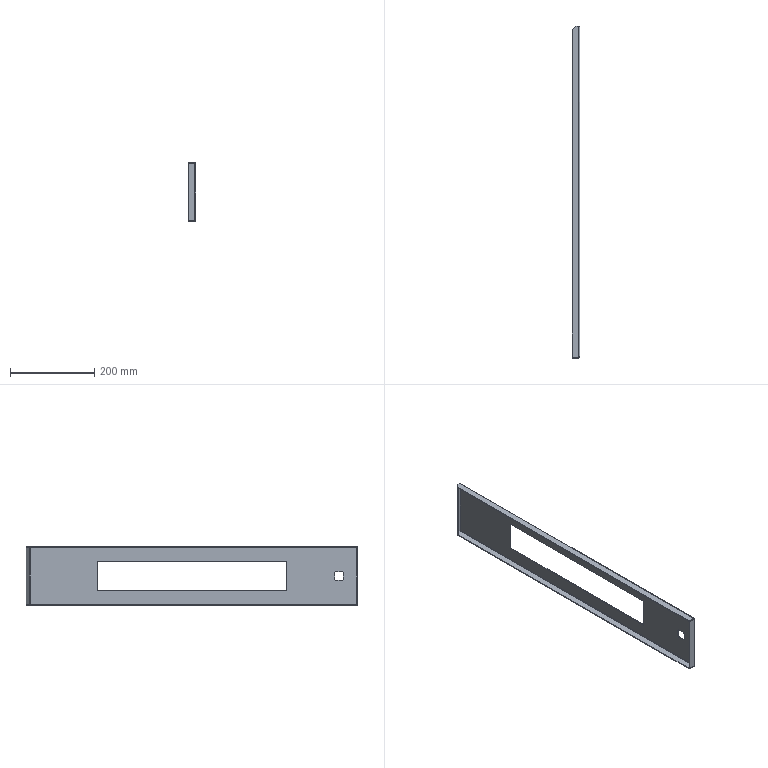Component | SolidWorks | FrontLowerDoor.2-1 | 1 solid | 67 faces | volume 213780 mm3 | plane 49 | cylinder 14 | spline 4 | commonest cylinder face diameters 6 x9 2 x5